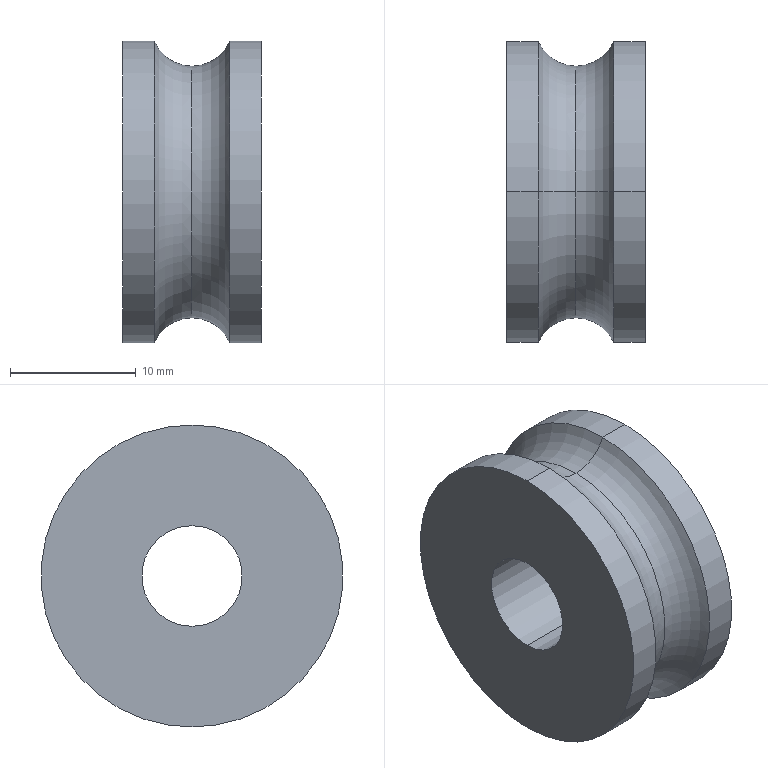Component | SolidWorks | U8-24-11SlotWidth6SlotDepth2-1 | 1 solid | 12 faces | box 11 x 24 x 24 mm | volume 3815 mm3 | cylinder 6 | torus 4 | plane 2 | commonest cylinder face diameters 24 x4 8 x2
build123d program:
from build123d import *


with BuildPart() as part:
    # Sketch1 → Revolve1 (revolve)
    with BuildSketch(Plane(origin=(0, 0, 0), x_dir=(0, 0, -1), z_dir=(1, 0, 0)), mode=Mode.PRIVATE) as revolve1_sk:
        with BuildLine():
            Line((-5.5, 12), (-3, 12))
            ThreePointArc((-3, 12), (0, 10), (3, 12))
            Line((3, 12), (5.5, 12))
            Line((5.5, 12), (5.5, 4))
            Line((5.5, 4), (-5.5, 4))
            Line((-5.5, 4), (-5.5, 12))
        make_face()
    revolve(revolve1_sk.sketch.rotate(Axis((0, 0, 29.232), (0, 0, -1)), 90), axis=Axis((0, 0, 29.232), (0, 0, -1)))


solid = part.part

# Placed as in the assembly
solid = solid.moved(Location((-237.5, 127.823, 79.212), (0, 90, 0)))
STEP:
#1=COLOUR_RGB('',0.7922,0.8196,0.9333);
#2=FILL_AREA_STYLE_COLOUR('',#1);
#3=FILL_AREA_STYLE('',(#2));
#4=SURFACE_STYLE_FILL_AREA(#3);
#5=SURFACE_SIDE_STYLE('',(#4));
#6=SURFACE_STYLE_USAGE(.BOTH.,#5);
#7=PRESENTATION_STYLE_ASSIGNMENT((#6));
#8=CARTESIAN_POINT('',(-9.469,5.032,3.591));
#9=VERTEX_POINT('',#8);
#10=CARTESIAN_POINT('',(-9.35,5.032,3.512));
#11=VERTEX_POINT('',#10);
#12=CARTESIAN_POINT('',(-9.35,5.032,3.64));
#13=DIRECTION('',(0.,-1.,0.));
#14=DIRECTION('',(0.,0.,-1.));
#15=AXIS2_PLACEMENT_3D('',#12,#13,#14);
#16=CIRCLE('',#15,0.128);
#17=EDGE_CURVE('',#9,#11,#16,.T.);
#18=ORIENTED_EDGE('',*,*,#17,.T.);
#19=CARTESIAN_POINT('',(-9.35,5.032,2.725));
#20=VERTEX_POINT('',#19);
#21=CARTESIAN_POINT('',(-9.35,5.032,3.119));
#22=DIRECTION('',(-1.,0.,0.));
#23=DIRECTION('',(0.,0.,1.));
#24=AXIS2_PLACEMENT_3D('',#21,#22,#23);
#25=CIRCLE('',#24,0.3937);
#26=EDGE_CURVE('',#11,#20,#25,.T.);
#27=ORIENTED_EDGE('',*,*,#26,.T.);
#28=CARTESIAN_POINT('',(-9.469,5.032,2.646));
#29=VERTEX_POINT('',#28);
#30=CARTESIAN_POINT('',(-9.35,5.032,2.597));
#31=DIRECTION('',(0.,1.,0.));
#32=DIRECTION('',(0.,0.,1.));
#33=AXIS2_PLACEMENT_3D('',#30,#31,#32);
#34=CIRCLE('',#33,0.128);
#35=EDGE_CURVE('',#29,#20,#34,.T.);
#36=ORIENTED_EDGE('',*,*,#35,.F.);
#37=CARTESIAN_POINT('',(-9.469,5.032,3.119));
#38=DIRECTION('',(-1.,0.,0.));
#39=DIRECTION('',(0.,0.,1.));
#40=AXIS2_PLACEMENT_3D('',#37,#38,#39);
#41=CIRCLE('',#40,0.4724);
#42=EDGE_CURVE('',#9,#29,#41,.T.);
#43=ORIENTED_EDGE('',*,*,#42,.F.);
#44=EDGE_LOOP('',(#18,#27,#36,#43));
#45=FACE_OUTER_BOUND('',#44,.T.);
#46=CARTESIAN_POINT('',(-9.35,5.032,3.119));
#47=DIRECTION('',(-1.,0.,0.));
#48=DIRECTION('',(0.,0.,1.));
#49=AXIS2_PLACEMENT_3D('',#46,#47,#48);
#50=TOROIDAL_SURFACE('',#49,0.5217,0.128);
#51=ADVANCED_FACE('',(#45),#50,.F.);
#52=ORIENTED_EDGE('',*,*,#35,.T.);
#53=CARTESIAN_POINT('',(-9.35,5.032,3.119));
#54=DIRECTION('',(-1.,0.,0.));
#55=DIRECTION('',(0.,0.,1.));
#56=AXIS2_PLACEMENT_3D('',#53,#54,#55);
#57=CIRCLE('',#56,0.3937);
#58=EDGE_CURVE('',#20,#11,#57,.T.);
#59=ORIENTED_EDGE('',*,*,#58,.T.);
#60=ORIENTED_EDGE('',*,*,#17,.F.);
#61=CARTESIAN_POINT('',(-9.469,5.032,3.119));
#62=DIRECTION('',(-1.,0.,0.));
#63=DIRECTION('',(0.,0.,1.));
#64=AXIS2_PLACEMENT_3D('',#61,#62,#63);
#65=CIRCLE('',#64,0.4724);
#66=EDGE_CURVE('',#29,#9,#65,.T.);
#67=ORIENTED_EDGE('',*,*,#66,.F.);
#68=EDGE_LOOP('',(#52,#59,#60,#67));
#69=FACE_OUTER_BOUND('',#68,.T.);
#70=CARTESIAN_POINT('',(-9.35,5.032,3.119));
#71=DIRECTION('',(-1.,0.,0.));
#72=DIRECTION('',(0.,0.,1.));
#73=AXIS2_PLACEMENT_3D('',#70,#71,#72);
#74=TOROIDAL_SURFACE('',#73,0.5217,0.128);
#75=ADVANCED_FACE('',(#69),#74,.F.);
#76=CARTESIAN_POINT('',(-9.134,5.032,2.961));
#77=VERTEX_POINT('',#76);
#78=CARTESIAN_POINT('',(-9.134,5.032,3.276));
#79=VERTEX_POINT('',#78);
#80=CARTESIAN_POINT('',(-9.134,5.032,3.119));
#81=DIRECTION('',(-1.,0.,0.));
#82=DIRECTION('',(0.,0.,1.));
#83=AXIS2_PLACEMENT_3D('',#80,#81,#82);
#84=CIRCLE('',#83,0.1575);
#85=EDGE_CURVE('',#77,#79,#84,.T.);
#86=ORIENTED_EDGE('',*,*,#85,.F.);
#87=CARTESIAN_POINT('',(-9.567,5.032,2.961));
#88=VERTEX_POINT('',#87);
#89=CARTESIAN_POINT('',(-10.501,5.032,2.961));
#90=DIRECTION('',(-1.,0.,0.));
#91=VECTOR('',#90,39.37);
#92=LINE('',#89,#91);
#93=EDGE_CURVE('',#77,#88,#92,.T.);
#94=ORIENTED_EDGE('',*,*,#93,.T.);
#95=CARTESIAN_POINT('',(-9.567,5.032,3.276));
#96=VERTEX_POINT('',#95);
#97=CARTESIAN_POINT('',(-9.567,5.032,3.119));
#98=DIRECTION('',(-1.,0.,0.));
#99=DIRECTION('',(0.,0.,1.));
#100=AXIS2_PLACEMENT_3D('',#97,#98,#99);
#101=CIRCLE('',#100,0.1575);
#102=EDGE_CURVE('',#88,#96,#101,.T.);
#103=ORIENTED_EDGE('',*,*,#102,.T.);
#104=CARTESIAN_POINT('',(-10.501,5.032,3.276));
#105=DIRECTION('',(-1.,0.,0.));
#106=VECTOR('',#105,39.37);
#107=LINE('',#104,#106);
#108=EDGE_CURVE('',#79,#96,#107,.T.);
#109=ORIENTED_EDGE('',*,*,#108,.F.);
#110=EDGE_LOOP('',(#86,#94,#103,#109));
#111=FACE_OUTER_BOUND('',#110,.T.);
#112=CARTESIAN_POINT('',(-10.501,5.032,3.119));
#113=DIRECTION('',(-1.,0.,0.));
#114=DIRECTION('',(0.,0.,1.));
#115=AXIS2_PLACEMENT_3D('',#112,#113,#114);
#116=CYLINDRICAL_SURFACE('',#115,0.1575);
#117=ADVANCED_FACE('',(#111),#116,.F.);
#118=ORIENTED_EDGE('',*,*,#42,.T.);
#119=CARTESIAN_POINT('',(-9.567,5.032,2.646));
#120=VERTEX_POINT('',#119);
#121=CARTESIAN_POINT('',(-10.501,5.032,2.646));
#122=DIRECTION('',(-1.,0.,0.));
#123=VECTOR('',#122,39.37);
#124=LINE('',#121,#123);
#125=EDGE_CURVE('',#29,#120,#124,.T.);
#126=ORIENTED_EDGE('',*,*,#125,.T.);
#127=CARTESIAN_POINT('',(-9.567,5.032,3.591));
#128=VERTEX_POINT('',#127);
#129=CARTESIAN_POINT('',(-9.567,5.032,3.119));
#130=DIRECTION('',(-1.,0.,0.));
#131=DIRECTION('',(0.,0.,1.));
#132=AXIS2_PLACEMENT_3D('',#129,#130,#131);
#133=CIRCLE('',#132,0.4724);
#134=EDGE_CURVE('',#128,#120,#133,.T.);
#135=ORIENTED_EDGE('',*,*,#134,.F.);
#136=CARTESIAN_POINT('',(-10.501,5.032,3.591));
#137=DIRECTION('',(-1.,0.,0.));
#138=VECTOR('',#137,39.37);
#139=LINE('',#136,#138);
#140=EDGE_CURVE('',#9,#128,#139,.T.);
#141=ORIENTED_EDGE('',*,*,#140,.F.);
#142=EDGE_LOOP('',(#118,#126,#135,#141));
#143=FACE_OUTER_BOUND('',#142,.T.);
#144=CARTESIAN_POINT('',(-10.501,5.032,3.119));
#145=DIRECTION('',(-1.,0.,0.));
#146=DIRECTION('',(0.,0.,1.));
#147=AXIS2_PLACEMENT_3D('',#144,#145,#146);
#148=CYLINDRICAL_SURFACE('',#147,0.4724);
#149=ADVANCED_FACE('',(#143),#148,.T.);
#150=ORIENTED_EDGE('',*,*,#58,.F.);
#151=CARTESIAN_POINT('',(-9.232,5.032,2.646));
#152=VERTEX_POINT('',#151);
#153=CARTESIAN_POINT('',(-9.35,5.032,2.597));
#154=DIRECTION('',(0.,1.,0.));
#155=DIRECTION('',(0.,0.,1.));
#156=AXIS2_PLACEMENT_3D('',#153,#154,#155);
#157=CIRCLE('',#156,0.128);
#158=EDGE_CURVE('',#20,#152,#157,.T.);
#159=ORIENTED_EDGE('',*,*,#158,.T.);
#160=CARTESIAN_POINT('',(-9.232,5.032,3.591));
#161=VERTEX_POINT('',#160);
#162=CARTESIAN_POINT('',(-9.232,5.032,3.119));
#163=DIRECTION('',(-1.,0.,0.));
#164=DIRECTION('',(0.,0.,1.));
#165=AXIS2_PLACEMENT_3D('',#162,#163,#164);
#166=CIRCLE('',#165,0.4724);
#167=EDGE_CURVE('',#152,#161,#166,.T.);
#168=ORIENTED_EDGE('',*,*,#167,.T.);
#169=CARTESIAN_POINT('',(-9.35,5.032,3.64));
#170=DIRECTION('',(0.,-1.,0.));
#171=DIRECTION('',(0.,0.,-1.));
#172=AXIS2_PLACEMENT_3D('',#169,#170,#171);
#173=CIRCLE('',#172,0.128);
#174=EDGE_CURVE('',#11,#161,#173,.T.);
#175=ORIENTED_EDGE('',*,*,#174,.F.);
#176=EDGE_LOOP('',(#150,#159,#168,#175));
#177=FACE_OUTER_BOUND('',#176,.T.);
#178=CARTESIAN_POINT('',(-9.35,5.032,3.119));
#179=DIRECTION('',(-1.,0.,0.));
#180=DIRECTION('',(0.,0.,1.));
#181=AXIS2_PLACEMENT_3D('',#178,#179,#180);
#182=TOROIDAL_SURFACE('',#181,0.5217,0.128);
#183=ADVANCED_FACE('',(#177),#182,.F.);
#184=CARTESIAN_POINT('',(-9.134,5.032,3.591));
#185=VERTEX_POINT('',#184);
#186=CARTESIAN_POINT('',(-9.134,5.032,2.646));
#187=VERTEX_POINT('',#186);
#188=CARTESIAN_POINT('',(-9.134,5.032,3.119));
#189=DIRECTION('',(-1.,0.,0.));
#190=DIRECTION('',(0.,0.,1.));
#191=AXIS2_PLACEMENT_3D('',#188,#189,#190);
#192=CIRCLE('',#191,0.4724);
#193=EDGE_CURVE('',#185,#187,#192,.T.);
#194=ORIENTED_EDGE('',*,*,#193,.T.);
#195=CARTESIAN_POINT('',(-10.501,5.032,2.646));
#196=DIRECTION('',(-1.,0.,0.));
#197=VECTOR('',#196,39.37);
#198=LINE('',#195,#197);
#199=EDGE_CURVE('',#187,#152,#198,.T.);
#200=ORIENTED_EDGE('',*,*,#199,.T.);
#201=CARTESIAN_POINT('',(-9.232,5.032,3.119));
#202=DIRECTION('',(-1.,0.,0.));
#203=DIRECTION('',(0.,0.,1.));
#204=AXIS2_PLACEMENT_3D('',#201,#202,#203);
#205=CIRCLE('',#204,0.4724);
#206=EDGE_CURVE('',#161,#152,#205,.T.);
#207=ORIENTED_EDGE('',*,*,#206,.F.);
#208=CARTESIAN_POINT('',(-10.501,5.032,3.591));
#209=DIRECTION('',(-1.,0.,0.));
#210=VECTOR('',#209,39.37);
#211=LINE('',#208,#210);
#212=EDGE_CURVE('',#185,#161,#211,.T.);
#213=ORIENTED_EDGE('',*,*,#212,.F.);
#214=EDGE_LOOP('',(#194,#200,#207,#213));
#215=FACE_OUTER_BOUND('',#214,.T.);
#216=CARTESIAN_POINT('',(-10.501,5.032,3.119));
#217=DIRECTION('',(-1.,0.,0.));
#218=DIRECTION('',(0.,0.,1.));
#219=AXIS2_PLACEMENT_3D('',#216,#217,#218);
#220=CYLINDRICAL_SURFACE('',#219,0.4724);
#221=ADVANCED_FACE('',(#215),#220,.T.);
#222=ORIENTED_EDGE('',*,*,#199,.F.);
#223=CARTESIAN_POINT('',(-9.134,5.032,3.119));
#224=DIRECTION('',(-1.,0.,0.));
#225=DIRECTION('',(0.,0.,1.));
#226=AXIS2_PLACEMENT_3D('',#223,#224,#225);
#227=CIRCLE('',#226,0.4724);
#228=EDGE_CURVE('',#187,#185,#227,.T.);
#229=ORIENTED_EDGE('',*,*,#228,.T.);
#230=ORIENTED_EDGE('',*,*,#212,.T.);
#231=ORIENTED_EDGE('',*,*,#167,.F.);
#232=EDGE_LOOP('',(#222,#229,#230,#231));
#233=FACE_OUTER_BOUND('',#232,.T.);
#234=CARTESIAN_POINT('',(-10.501,5.032,3.119));
#235=DIRECTION('',(-1.,0.,0.));
#236=DIRECTION('',(0.,0.,1.));
#237=AXIS2_PLACEMENT_3D('',#234,#235,#236);
#238=CYLINDRICAL_SURFACE('',#237,0.4724);
#239=ADVANCED_FACE('',(#233),#238,.T.);
#240=ORIENTED_EDGE('',*,*,#26,.F.);
#241=ORIENTED_EDGE('',*,*,#174,.T.);
#242=ORIENTED_EDGE('',*,*,#206,.T.);
#243=ORIENTED_EDGE('',*,*,#158,.F.);
#244=EDGE_LOOP('',(#240,#241,#242,#243));
#245=FACE_OUTER_BOUND('',#244,.T.);
#246=CARTESIAN_POINT('',(-9.35,5.032,3.119));
#247=DIRECTION('',(-1.,0.,0.));
#248=DIRECTION('',(0.,0.,1.));
#249=AXIS2_PLACEMENT_3D('',#246,#247,#248);
#250=TOROIDAL_SURFACE('',#249,0.5217,0.128);
#251=ADVANCED_FACE('',(#245),#250,.F.);
#252=ORIENTED_EDGE('',*,*,#125,.F.);
#253=ORIENTED_EDGE('',*,*,#66,.T.);
#254=ORIENTED_EDGE('',*,*,#140,.T.);
#255=CARTESIAN_POINT('',(-9.567,5.032,3.119));
#256=DIRECTION('',(-1.,0.,0.));
#257=DIRECTION('',(0.,0.,1.));
#258=AXIS2_PLACEMENT_3D('',#255,#256,#257);
#259=CIRCLE('',#258,0.4724);
#260=EDGE_CURVE('',#120,#128,#259,.T.);
#261=ORIENTED_EDGE('',*,*,#260,.F.);
#262=EDGE_LOOP('',(#252,#253,#254,#261));
#263=FACE_OUTER_BOUND('',#262,.T.);
#264=CARTESIAN_POINT('',(-10.501,5.032,3.119));
#265=DIRECTION('',(-1.,0.,0.));
#266=DIRECTION('',(0.,0.,1.));
#267=AXIS2_PLACEMENT_3D('',#264,#265,#266);
#268=CYLINDRICAL_SURFACE('',#267,0.4724);
#269=ADVANCED_FACE('',(#263),#268,.T.);
#270=CARTESIAN_POINT('',(-9.567,5.032,3.119));
#271=DIRECTION('',(-1.,0.,0.));
#272=DIRECTION('',(0.,0.,1.));
#273=AXIS2_PLACEMENT_3D('',#270,#271,#272);
#274=CIRCLE('',#273,0.1575);
#275=EDGE_CURVE('',#96,#88,#274,.T.);
#276=ORIENTED_EDGE('',*,*,#275,.F.);
#277=ORIENTED_EDGE('',*,*,#102,.F.);
#278=EDGE_LOOP('',(#276,#277));
#279=FACE_BOUND('',#278,.T.);
#280=ORIENTED_EDGE('',*,*,#134,.T.);
#281=ORIENTED_EDGE('',*,*,#260,.T.);
#282=EDGE_LOOP('',(#280,#281));
#283=FACE_OUTER_BOUND('',#282,.T.);
#284=CARTESIAN_POINT('',(-9.567,5.505,3.119));
#285=DIRECTION('',(1.,0.,0.));
#286=DIRECTION('',(0.,0.,-1.));
#287=AXIS2_PLACEMENT_3D('',#284,#285,#286);
#288=PLANE('',#287);
#289=ADVANCED_FACE('',(#279,#283),#288,.F.);
#290=ORIENTED_EDGE('',*,*,#93,.F.);
#291=CARTESIAN_POINT('',(-9.134,5.032,3.119));
#292=DIRECTION('',(-1.,0.,0.));
#293=DIRECTION('',(0.,0.,1.));
#294=AXIS2_PLACEMENT_3D('',#291,#292,#293);
#295=CIRCLE('',#294,0.1575);
#296=EDGE_CURVE('',#79,#77,#295,.T.);
#297=ORIENTED_EDGE('',*,*,#296,.F.);
#298=ORIENTED_EDGE('',*,*,#108,.T.);
#299=ORIENTED_EDGE('',*,*,#275,.T.);
#300=EDGE_LOOP('',(#290,#297,#298,#299));
#301=FACE_OUTER_BOUND('',#300,.T.);
#302=CARTESIAN_POINT('',(-10.501,5.032,3.119));
#303=DIRECTION('',(-1.,0.,0.));
#304=DIRECTION('',(0.,0.,1.));
#305=AXIS2_PLACEMENT_3D('',#302,#303,#304);
#306=CYLINDRICAL_SURFACE('',#305,0.1575);
#307=ADVANCED_FACE('',(#301),#306,.F.);
#308=ORIENTED_EDGE('',*,*,#193,.F.);
#309=ORIENTED_EDGE('',*,*,#228,.F.);
#310=EDGE_LOOP('',(#308,#309));
#311=FACE_OUTER_BOUND('',#310,.T.);
#312=ORIENTED_EDGE('',*,*,#296,.T.);
#313=ORIENTED_EDGE('',*,*,#85,.T.);
#314=EDGE_LOOP('',(#312,#313));
#315=FACE_BOUND('',#314,.T.);
#316=CARTESIAN_POINT('',(-9.134,5.505,3.119));
#317=DIRECTION('',(-1.,0.,0.));
#318=DIRECTION('',(0.,0.,1.));
#319=AXIS2_PLACEMENT_3D('',#316,#317,#318);
#320=PLANE('',#319);
#321=ADVANCED_FACE('',(#311,#315),#320,.F.);
#322=CLOSED_SHELL('',(#51,#75,#117,#149,#183,#221,#239,#251,#269,#289,#307,#321));
#323=MANIFOLD_SOLID_BREP('',#322);
#324=STYLED_ITEM('',(#7),#323);
#325=PRESENTATION_LAYER_ASSIGNMENT('','',(#324));
#326=(LENGTH_UNIT()NAMED_UNIT(*)SI_UNIT($,.METRE.));
#327=LENGTH_MEASURE_WITH_UNIT(LENGTH_MEASURE(0.0254),#326);
#328=DIMENSIONAL_EXPONENTS(1.,0.,0.,0.,0.,0.,0.);
#329=(CONVERSION_BASED_UNIT('',#327)LENGTH_UNIT()NAMED_UNIT(#328));
#330=UNCERTAINTY_MEASURE_WITH_UNIT(LENGTH_MEASURE(0.00001),#329,'','');
#331=(NAMED_UNIT(*)PLANE_ANGLE_UNIT()SI_UNIT($,.RADIAN.));
#332=(NAMED_UNIT(*)SI_UNIT($,.STERADIAN.)SOLID_ANGLE_UNIT());
#333=(GEOMETRIC_REPRESENTATION_CONTEXT(3)GLOBAL_UNCERTAINTY_ASSIGNED_CONTEXT((#330))GLOBAL_UNIT_ASSIGNED_CONTEXT((#329,#331,#332))REPRESENTATION_CONTEXT('',''));
#334=MECHANICAL_DESIGN_GEOMETRIC_PRESENTATION_REPRESENTATION('',(#324),#333);
#335=CARTESIAN_POINT('',(0.,0.,0.));
#336=DIRECTION('',(0.,0.,1.));
#337=DIRECTION('',(1.,0.,0.));
#338=AXIS2_PLACEMENT_3D('',#335,#336,#337);
#339=(LENGTH_UNIT()NAMED_UNIT(*)SI_UNIT($,.METRE.));
#340=LENGTH_MEASURE_WITH_UNIT(LENGTH_MEASURE(0.0254),#339);
#341=DIMENSIONAL_EXPONENTS(1.,0.,0.,0.,0.,0.,0.);
#342=(CONVERSION_BASED_UNIT('',#340)LENGTH_UNIT()NAMED_UNIT(#341));
#343=UNCERTAINTY_MEASURE_WITH_UNIT(LENGTH_MEASURE(0.00001),#342,'','');
#344=(NAMED_UNIT(*)PLANE_ANGLE_UNIT()SI_UNIT($,.RADIAN.));
#345=(NAMED_UNIT(*)SI_UNIT($,.STERADIAN.)SOLID_ANGLE_UNIT());
#346=(GEOMETRIC_REPRESENTATION_CONTEXT(3)GLOBAL_UNCERTAINTY_ASSIGNED_CONTEXT((#343))GLOBAL_UNIT_ASSIGNED_CONTEXT((#342,#344,#345))REPRESENTATION_CONTEXT('',''));
#347=ADVANCED_BREP_SHAPE_REPRESENTATION('',(#323,#338),#346);